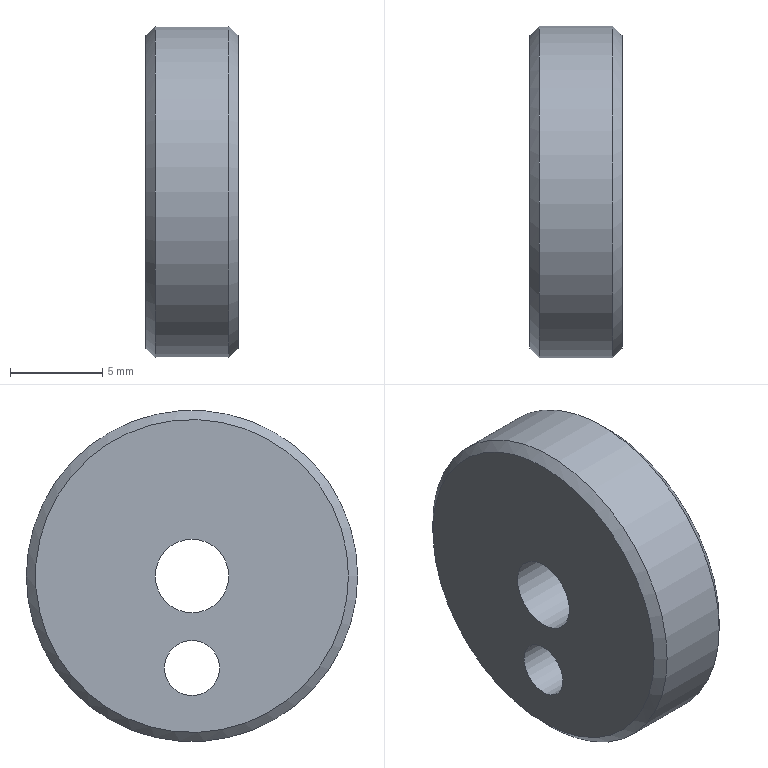Component | NX | ASSY_PRAC_PART_3 | 1 solid | 7 faces | box 5 x 18 x 18 mm | volume 1160 mm3 | cylinder 3 | plane 2 | cone 2 | commonest cylinder face diameters 3 x1 18 x1 4 x1
STEP:
#1=CARTESIAN_POINT('',(0.,0.,0.));
#2=DIRECTION('',(0.,0.,1.));
#3=DIRECTION('',(1.,0.,0.));
#4=AXIS2_PLACEMENT_3D('',#1,#2,#3);
#5=CARTESIAN_POINT('',(-8.5,-1.115,15.561));
#6=VERTEX_POINT('',#5);
#7=CARTESIAN_POINT('',(-8.5,0.3851,15.561));
#8=DIRECTION('',(-1.,0.,0.));
#9=DIRECTION('',(0.,-1.,0.));
#10=AXIS2_PLACEMENT_3D('',#7,#8,#9);
#11=CIRCLE('',#10,1.5);
#12=CARTESIAN_POINT('',(-8.5,0.3851,15.561));
#13=DIRECTION('',(-1.,0.,0.));
#14=DIRECTION('',(0.,1.,0.));
#15=AXIS2_PLACEMENT_3D('',#12,#13,#14);
#16=CYLINDRICAL_SURFACE('',#15,1.5);
#17=CARTESIAN_POINT('',(3.142,0.));
#18=DIRECTION('',(1.,0.));
#19=VECTOR('',#18,1.);
#20=LINE('',#17,#19);
#21=(GEOMETRIC_REPRESENTATION_CONTEXT(2)PARAMETRIC_REPRESENTATION_CONTEXT()REPRESENTATION_CONTEXT('',''));
#22=DEFINITIONAL_REPRESENTATION('',(#20),#21);
#23=PCURVE('',#16,#22);
#24=CARTESIAN_POINT('',(-8.5,0.3851,18.061));
#25=DIRECTION('',(1.,0.,0.));
#26=DIRECTION('',(0.,-1.,0.));
#27=AXIS2_PLACEMENT_3D('',#24,#25,#26);
#28=PLANE('',#27);
#29=CARTESIAN_POINT('',(1.5,2.5));
#30=CARTESIAN_POINT('',(1.5,-0.09808));
#31=CARTESIAN_POINT('',(-0.75,1.201));
#32=CARTESIAN_POINT('',(-3.,2.5));
#33=CARTESIAN_POINT('',(-0.75,3.799));
#34=CARTESIAN_POINT('',(1.5,5.098));
#35=CARTESIAN_POINT('',(1.5,2.5));
#36=(BOUNDED_CURVE()B_SPLINE_CURVE(2,(#29,#30,#31,#32,#33,#34,#35),.UNSPECIFIED.,.T.,.F.)B_SPLINE_CURVE_WITH_KNOTS((1,2,2,2,2,1),(-2.094,0.,2.094,4.189,6.283,8.378),.UNSPECIFIED.)CURVE()GEOMETRIC_REPRESENTATION_ITEM()RATIONAL_B_SPLINE_CURVE((1.,0.5,1.,0.5,1.,0.5,1.))REPRESENTATION_ITEM(''));
#37=(GEOMETRIC_REPRESENTATION_CONTEXT(2)PARAMETRIC_REPRESENTATION_CONTEXT()REPRESENTATION_CONTEXT('',''));
#38=DEFINITIONAL_REPRESENTATION('',(#36),#37);
#39=PCURVE('',#28,#38);
#40=SURFACE_CURVE('',#11,(#23,#39),.PCURVE_S1.);
#41=EDGE_CURVE('',#6,#6,#40,.T.);
#42=ORIENTED_EDGE('',*,*,#41,.T.);
#43=CARTESIAN_POINT('',(-13.5,-1.115,15.561));
#44=VERTEX_POINT('',#43);
#45=CARTESIAN_POINT('',(-8.5,-1.115,15.561));
#46=CARTESIAN_POINT('',(-13.5,-1.115,15.561));
#47=B_SPLINE_CURVE_WITH_KNOTS('',1,(#45,#46),.UNSPECIFIED.,.F.,.F.,(2,2),(0.,5.),.PIECEWISE_BEZIER_KNOTS.);
#48=CARTESIAN_POINT('',(9.425,0.));
#49=DIRECTION('',(0.,1.));
#50=VECTOR('',#49,1.);
#51=LINE('',#48,#50);
#52=(GEOMETRIC_REPRESENTATION_CONTEXT(2)PARAMETRIC_REPRESENTATION_CONTEXT()REPRESENTATION_CONTEXT('',''));
#53=DEFINITIONAL_REPRESENTATION('',(#51),#52);
#54=PCURVE('',#16,#53);
#55=CARTESIAN_POINT('',(3.142,0.));
#56=DIRECTION('',(0.,1.));
#57=VECTOR('',#56,1.);
#58=LINE('',#55,#57);
#59=(GEOMETRIC_REPRESENTATION_CONTEXT(2)PARAMETRIC_REPRESENTATION_CONTEXT()REPRESENTATION_CONTEXT('',''));
#60=DEFINITIONAL_REPRESENTATION('',(#58),#59);
#61=PCURVE('',#16,#60);
#62=SEAM_CURVE('',#47,(#54,#61),.PCURVE_S1.);
#63=EDGE_CURVE('',#6,#44,#62,.T.);
#64=ORIENTED_EDGE('',*,*,#63,.T.);
#65=CARTESIAN_POINT('',(-13.5,0.3851,15.561));
#66=DIRECTION('',(-1.,0.,0.));
#67=DIRECTION('',(0.,-1.,0.));
#68=AXIS2_PLACEMENT_3D('',#65,#66,#67);
#69=CIRCLE('',#68,1.5);
#70=CARTESIAN_POINT('',(3.142,5.));
#71=DIRECTION('',(1.,0.));
#72=VECTOR('',#71,1.);
#73=LINE('',#70,#72);
#74=(GEOMETRIC_REPRESENTATION_CONTEXT(2)PARAMETRIC_REPRESENTATION_CONTEXT()REPRESENTATION_CONTEXT('',''));
#75=DEFINITIONAL_REPRESENTATION('',(#73),#74);
#76=PCURVE('',#16,#75);
#77=CARTESIAN_POINT('',(-13.5,0.3851,18.061));
#78=DIRECTION('',(1.,0.,0.));
#79=DIRECTION('',(0.,-1.,0.));
#80=AXIS2_PLACEMENT_3D('',#77,#78,#79);
#81=PLANE('',#80);
#82=CARTESIAN_POINT('',(1.5,2.5));
#83=CARTESIAN_POINT('',(1.5,-0.09808));
#84=CARTESIAN_POINT('',(-0.75,1.201));
#85=CARTESIAN_POINT('',(-3.,2.5));
#86=CARTESIAN_POINT('',(-0.75,3.799));
#87=CARTESIAN_POINT('',(1.5,5.098));
#88=CARTESIAN_POINT('',(1.5,2.5));
#89=(BOUNDED_CURVE()B_SPLINE_CURVE(2,(#82,#83,#84,#85,#86,#87,#88),.UNSPECIFIED.,.T.,.F.)B_SPLINE_CURVE_WITH_KNOTS((1,2,2,2,2,1),(-2.094,0.,2.094,4.189,6.283,8.378),.UNSPECIFIED.)CURVE()GEOMETRIC_REPRESENTATION_ITEM()RATIONAL_B_SPLINE_CURVE((1.,0.5,1.,0.5,1.,0.5,1.))REPRESENTATION_ITEM(''));
#90=(GEOMETRIC_REPRESENTATION_CONTEXT(2)PARAMETRIC_REPRESENTATION_CONTEXT()REPRESENTATION_CONTEXT('',''));
#91=DEFINITIONAL_REPRESENTATION('',(#89),#90);
#92=PCURVE('',#81,#91);
#93=SURFACE_CURVE('',#69,(#76,#92),.PCURVE_S1.);
#94=EDGE_CURVE('',#44,#44,#93,.T.);
#95=ORIENTED_EDGE('',*,*,#94,.F.);
#96=ORIENTED_EDGE('',*,*,#63,.F.);
#97=EDGE_LOOP('',(#42,#64,#95,#96));
#98=FACE_BOUND('',#97,.F.);
#99=ADVANCED_FACE('',(#98),#16,.F.);
#100=CARTESIAN_POINT('',(-13.,-8.615,20.561));
#101=VERTEX_POINT('',#100);
#102=CARTESIAN_POINT('',(-13.,0.3851,20.561));
#103=DIRECTION('',(1.,0.,0.));
#104=DIRECTION('',(0.,-1.,0.));
#105=AXIS2_PLACEMENT_3D('',#102,#103,#104);
#106=CIRCLE('',#105,9.);
#107=CARTESIAN_POINT('',(-8.5,0.3851,20.561));
#108=DIRECTION('',(-1.,0.,0.));
#109=DIRECTION('',(0.,1.,0.));
#110=AXIS2_PLACEMENT_3D('',#107,#108,#109);
#111=CYLINDRICAL_SURFACE('',#110,9.);
#112=CARTESIAN_POINT('',(9.425,4.5));
#113=DIRECTION('',(-1.,0.));
#114=VECTOR('',#113,1.);
#115=LINE('',#112,#114);
#116=(GEOMETRIC_REPRESENTATION_CONTEXT(2)PARAMETRIC_REPRESENTATION_CONTEXT()REPRESENTATION_CONTEXT('',''));
#117=DEFINITIONAL_REPRESENTATION('',(#115),#116);
#118=PCURVE('',#111,#117);
#119=CARTESIAN_POINT('',(-13.5,0.3851,20.561));
#120=DIRECTION('',(1.,0.,0.));
#121=DIRECTION('',(0.,-1.,0.));
#122=AXIS2_PLACEMENT_3D('',#119,#120,#121);
#123=CONICAL_SURFACE('',#122,8.5,0.7854);
#124=CARTESIAN_POINT('',(0.,0.5));
#125=DIRECTION('',(1.,0.));
#126=VECTOR('',#125,1.);
#127=LINE('',#124,#126);
#128=(GEOMETRIC_REPRESENTATION_CONTEXT(2)PARAMETRIC_REPRESENTATION_CONTEXT()REPRESENTATION_CONTEXT('',''));
#129=DEFINITIONAL_REPRESENTATION('',(#127),#128);
#130=PCURVE('',#123,#129);
#131=SURFACE_CURVE('',#106,(#118,#130),.PCURVE_S1.);
#132=EDGE_CURVE('',#101,#101,#131,.T.);
#133=ORIENTED_EDGE('',*,*,#132,.T.);
#134=CARTESIAN_POINT('',(-9.,-8.615,20.561));
#135=VERTEX_POINT('',#134);
#136=CARTESIAN_POINT('',(-9.,-8.615,20.561));
#137=CARTESIAN_POINT('',(-13.,-8.615,20.561));
#138=B_SPLINE_CURVE_WITH_KNOTS('',1,(#136,#137),.UNSPECIFIED.,.F.,.F.,(2,2),(0.5,4.5),.PIECEWISE_BEZIER_KNOTS.);
#139=CARTESIAN_POINT('',(3.142,0.));
#140=DIRECTION('',(0.,1.));
#141=VECTOR('',#140,1.);
#142=LINE('',#139,#141);
#143=(GEOMETRIC_REPRESENTATION_CONTEXT(2)PARAMETRIC_REPRESENTATION_CONTEXT()REPRESENTATION_CONTEXT('',''));
#144=DEFINITIONAL_REPRESENTATION('',(#142),#143);
#145=PCURVE('',#111,#144);
#146=CARTESIAN_POINT('',(9.425,0.));
#147=DIRECTION('',(0.,1.));
#148=VECTOR('',#147,1.);
#149=LINE('',#146,#148);
#150=(GEOMETRIC_REPRESENTATION_CONTEXT(2)PARAMETRIC_REPRESENTATION_CONTEXT()REPRESENTATION_CONTEXT('',''));
#151=DEFINITIONAL_REPRESENTATION('',(#149),#150);
#152=PCURVE('',#111,#151);
#153=SEAM_CURVE('',#138,(#145,#152),.PCURVE_S1.);
#154=EDGE_CURVE('',#135,#101,#153,.T.);
#155=ORIENTED_EDGE('',*,*,#154,.F.);
#156=CARTESIAN_POINT('',(-9.,0.3851,20.561));
#157=DIRECTION('',(-1.,0.,0.));
#158=DIRECTION('',(0.,-1.,0.));
#159=AXIS2_PLACEMENT_3D('',#156,#157,#158);
#160=CIRCLE('',#159,9.);
#161=CARTESIAN_POINT('',(3.142,0.5));
#162=DIRECTION('',(1.,0.));
#163=VECTOR('',#162,1.);
#164=LINE('',#161,#163);
#165=(GEOMETRIC_REPRESENTATION_CONTEXT(2)PARAMETRIC_REPRESENTATION_CONTEXT()REPRESENTATION_CONTEXT('',''));
#166=DEFINITIONAL_REPRESENTATION('',(#164),#165);
#167=PCURVE('',#111,#166);
#168=CARTESIAN_POINT('',(-9.,0.3851,20.561));
#169=DIRECTION('',(-1.,0.,0.));
#170=DIRECTION('',(0.,1.,0.));
#171=AXIS2_PLACEMENT_3D('',#168,#169,#170);
#172=CONICAL_SURFACE('',#171,9.,0.7854);
#173=CARTESIAN_POINT('',(3.142,0.));
#174=DIRECTION('',(1.,0.));
#175=VECTOR('',#174,1.);
#176=LINE('',#173,#175);
#177=(GEOMETRIC_REPRESENTATION_CONTEXT(2)PARAMETRIC_REPRESENTATION_CONTEXT()REPRESENTATION_CONTEXT('',''));
#178=DEFINITIONAL_REPRESENTATION('',(#176),#177);
#179=PCURVE('',#172,#178);
#180=SURFACE_CURVE('',#160,(#167,#179),.PCURVE_S1.);
#181=EDGE_CURVE('',#135,#135,#180,.T.);
#182=ORIENTED_EDGE('',*,*,#181,.T.);
#183=ORIENTED_EDGE('',*,*,#154,.T.);
#184=EDGE_LOOP('',(#133,#155,#182,#183));
#185=FACE_BOUND('',#184,.T.);
#186=ADVANCED_FACE('',(#185),#111,.T.);
#187=CARTESIAN_POINT('',(-8.5,-1.615,20.561));
#188=VERTEX_POINT('',#187);
#189=CARTESIAN_POINT('',(-8.5,0.3851,20.561));
#190=DIRECTION('',(-1.,0.,0.));
#191=DIRECTION('',(0.,-1.,0.));
#192=AXIS2_PLACEMENT_3D('',#189,#190,#191);
#193=CIRCLE('',#192,2.);
#194=CARTESIAN_POINT('',(-8.5,0.3851,20.561));
#195=DIRECTION('',(-1.,0.,0.));
#196=DIRECTION('',(0.,1.,0.));
#197=AXIS2_PLACEMENT_3D('',#194,#195,#196);
#198=CYLINDRICAL_SURFACE('',#197,2.);
#199=CARTESIAN_POINT('',(3.142,0.));
#200=DIRECTION('',(1.,0.));
#201=VECTOR('',#200,1.);
#202=LINE('',#199,#201);
#203=(GEOMETRIC_REPRESENTATION_CONTEXT(2)PARAMETRIC_REPRESENTATION_CONTEXT()REPRESENTATION_CONTEXT('',''));
#204=DEFINITIONAL_REPRESENTATION('',(#202),#203);
#205=PCURVE('',#198,#204);
#206=CARTESIAN_POINT('',(2.,-2.5));
#207=CARTESIAN_POINT('',(2.,-5.964));
#208=CARTESIAN_POINT('',(-1.,-4.232));
#209=CARTESIAN_POINT('',(-4.,-2.5));
#210=CARTESIAN_POINT('',(-1.,-0.7679));
#211=CARTESIAN_POINT('',(2.,0.9641));
#212=CARTESIAN_POINT('',(2.,-2.5));
#213=(BOUNDED_CURVE()B_SPLINE_CURVE(2,(#206,#207,#208,#209,#210,#211,#212),.UNSPECIFIED.,.T.,.F.)B_SPLINE_CURVE_WITH_KNOTS((1,2,2,2,2,1),(-2.094,0.,2.094,4.189,6.283,8.378),.UNSPECIFIED.)CURVE()GEOMETRIC_REPRESENTATION_ITEM()RATIONAL_B_SPLINE_CURVE((1.,0.5,1.,0.5,1.,0.5,1.))REPRESENTATION_ITEM(''));
#214=(GEOMETRIC_REPRESENTATION_CONTEXT(2)PARAMETRIC_REPRESENTATION_CONTEXT()REPRESENTATION_CONTEXT('',''));
#215=DEFINITIONAL_REPRESENTATION('',(#213),#214);
#216=PCURVE('',#28,#215);
#217=SURFACE_CURVE('',#193,(#205,#216),.PCURVE_S1.);
#218=EDGE_CURVE('',#188,#188,#217,.T.);
#219=ORIENTED_EDGE('',*,*,#218,.T.);
#220=CARTESIAN_POINT('',(-13.5,-1.615,20.561));
#221=VERTEX_POINT('',#220);
#222=CARTESIAN_POINT('',(-8.5,-1.615,20.561));
#223=CARTESIAN_POINT('',(-13.5,-1.615,20.561));
#224=B_SPLINE_CURVE_WITH_KNOTS('',1,(#222,#223),.UNSPECIFIED.,.F.,.F.,(2,2),(0.,5.),.PIECEWISE_BEZIER_KNOTS.);
#225=CARTESIAN_POINT('',(9.425,0.));
#226=DIRECTION('',(0.,1.));
#227=VECTOR('',#226,1.);
#228=LINE('',#225,#227);
#229=(GEOMETRIC_REPRESENTATION_CONTEXT(2)PARAMETRIC_REPRESENTATION_CONTEXT()REPRESENTATION_CONTEXT('',''));
#230=DEFINITIONAL_REPRESENTATION('',(#228),#229);
#231=PCURVE('',#198,#230);
#232=CARTESIAN_POINT('',(3.142,0.));
#233=DIRECTION('',(0.,1.));
#234=VECTOR('',#233,1.);
#235=LINE('',#232,#234);
#236=(GEOMETRIC_REPRESENTATION_CONTEXT(2)PARAMETRIC_REPRESENTATION_CONTEXT()REPRESENTATION_CONTEXT('',''));
#237=DEFINITIONAL_REPRESENTATION('',(#235),#236);
#238=PCURVE('',#198,#237);
#239=SEAM_CURVE('',#224,(#231,#238),.PCURVE_S1.);
#240=EDGE_CURVE('',#188,#221,#239,.T.);
#241=ORIENTED_EDGE('',*,*,#240,.T.);
#242=CARTESIAN_POINT('',(-13.5,0.3851,20.561));
#243=DIRECTION('',(-1.,0.,0.));
#244=DIRECTION('',(0.,-1.,0.));
#245=AXIS2_PLACEMENT_3D('',#242,#243,#244);
#246=CIRCLE('',#245,2.);
#247=CARTESIAN_POINT('',(3.142,5.));
#248=DIRECTION('',(1.,0.));
#249=VECTOR('',#248,1.);
#250=LINE('',#247,#249);
#251=(GEOMETRIC_REPRESENTATION_CONTEXT(2)PARAMETRIC_REPRESENTATION_CONTEXT()REPRESENTATION_CONTEXT('',''));
#252=DEFINITIONAL_REPRESENTATION('',(#250),#251);
#253=PCURVE('',#198,#252);
#254=CARTESIAN_POINT('',(2.,-2.5));
#255=CARTESIAN_POINT('',(2.,-5.964));
#256=CARTESIAN_POINT('',(-1.,-4.232));
#257=CARTESIAN_POINT('',(-4.,-2.5));
#258=CARTESIAN_POINT('',(-1.,-0.7679));
#259=CARTESIAN_POINT('',(2.,0.9641));
#260=CARTESIAN_POINT('',(2.,-2.5));
#261=(BOUNDED_CURVE()B_SPLINE_CURVE(2,(#254,#255,#256,#257,#258,#259,#260),.UNSPECIFIED.,.T.,.F.)B_SPLINE_CURVE_WITH_KNOTS((1,2,2,2,2,1),(-2.094,0.,2.094,4.189,6.283,8.378),.UNSPECIFIED.)CURVE()GEOMETRIC_REPRESENTATION_ITEM()RATIONAL_B_SPLINE_CURVE((1.,0.5,1.,0.5,1.,0.5,1.))REPRESENTATION_ITEM(''));
#262=(GEOMETRIC_REPRESENTATION_CONTEXT(2)PARAMETRIC_REPRESENTATION_CONTEXT()REPRESENTATION_CONTEXT('',''));
#263=DEFINITIONAL_REPRESENTATION('',(#261),#262);
#264=PCURVE('',#81,#263);
#265=SURFACE_CURVE('',#246,(#253,#264),.PCURVE_S1.);
#266=EDGE_CURVE('',#221,#221,#265,.T.);
#267=ORIENTED_EDGE('',*,*,#266,.F.);
#268=ORIENTED_EDGE('',*,*,#240,.F.);
#269=EDGE_LOOP('',(#219,#241,#267,#268));
#270=FACE_BOUND('',#269,.F.);
#271=ADVANCED_FACE('',(#270),#198,.F.);
#272=CARTESIAN_POINT('',(-8.5,-8.115,20.561));
#273=VERTEX_POINT('',#272);
#274=CARTESIAN_POINT('',(-8.5,0.3851,20.561));
#275=DIRECTION('',(1.,0.,0.));
#276=DIRECTION('',(0.,-1.,0.));
#277=AXIS2_PLACEMENT_3D('',#274,#275,#276);
#278=CIRCLE('',#277,8.5);
#279=CARTESIAN_POINT('',(0.,-2.5));
#280=DIRECTION('',(1.,0.));
#281=AXIS2_PLACEMENT_2D('',#279,#280);
#282=CIRCLE('',#281,8.5);
#283=(GEOMETRIC_REPRESENTATION_CONTEXT(2)PARAMETRIC_REPRESENTATION_CONTEXT()REPRESENTATION_CONTEXT('',''));
#284=DEFINITIONAL_REPRESENTATION('',(#282),#283);
#285=PCURVE('',#28,#284);
#286=CARTESIAN_POINT('',(9.425,-0.5));
#287=DIRECTION('',(-1.,0.));
#288=VECTOR('',#287,1.);
#289=LINE('',#286,#288);
#290=(GEOMETRIC_REPRESENTATION_CONTEXT(2)PARAMETRIC_REPRESENTATION_CONTEXT()REPRESENTATION_CONTEXT('',''));
#291=DEFINITIONAL_REPRESENTATION('',(#289),#290);
#292=PCURVE('',#172,#291);
#293=SURFACE_CURVE('',#278,(#285,#292),.PCURVE_S1.);
#294=EDGE_CURVE('',#273,#273,#293,.T.);
#295=ORIENTED_EDGE('',*,*,#294,.T.);
#296=EDGE_LOOP('',(#295));
#297=FACE_BOUND('',#296,.T.);
#298=ORIENTED_EDGE('',*,*,#41,.T.);
#299=EDGE_LOOP('',(#298));
#300=FACE_BOUND('',#299,.T.);
#301=ORIENTED_EDGE('',*,*,#218,.T.);
#302=EDGE_LOOP('',(#301));
#303=FACE_BOUND('',#302,.T.);
#304=ADVANCED_FACE('',(#297,#300,#303),#28,.T.);
#305=CARTESIAN_POINT('',(-13.5,-8.115,20.561));
#306=VERTEX_POINT('',#305);
#307=CARTESIAN_POINT('',(-13.5,0.3851,20.561));
#308=DIRECTION('',(-1.,0.,0.));
#309=DIRECTION('',(0.,-1.,0.));
#310=AXIS2_PLACEMENT_3D('',#307,#308,#309);
#311=CIRCLE('',#310,8.5);
#312=CARTESIAN_POINT('',(8.5,-2.5));
#313=CARTESIAN_POINT('',(8.5,-17.222));
#314=CARTESIAN_POINT('',(-4.25,-9.861));
#315=CARTESIAN_POINT('',(-17.,-2.5));
#316=CARTESIAN_POINT('',(-4.25,4.861));
#317=CARTESIAN_POINT('',(8.5,12.222));
#318=CARTESIAN_POINT('',(8.5,-2.5));
#319=(BOUNDED_CURVE()B_SPLINE_CURVE(2,(#312,#313,#314,#315,#316,#317,#318),.UNSPECIFIED.,.T.,.F.)B_SPLINE_CURVE_WITH_KNOTS((1,2,2,2,2,1),(-2.094,0.,2.094,4.189,6.283,8.378),.UNSPECIFIED.)CURVE()GEOMETRIC_REPRESENTATION_ITEM()RATIONAL_B_SPLINE_CURVE((1.,0.5,1.,0.5,1.,0.5,1.))REPRESENTATION_ITEM(''));
#320=(GEOMETRIC_REPRESENTATION_CONTEXT(2)PARAMETRIC_REPRESENTATION_CONTEXT()REPRESENTATION_CONTEXT('',''));
#321=DEFINITIONAL_REPRESENTATION('',(#319),#320);
#322=PCURVE('',#81,#321);
#323=CARTESIAN_POINT('',(6.283,0.));
#324=DIRECTION('',(-1.,0.));
#325=VECTOR('',#324,1.);
#326=LINE('',#323,#325);
#327=(GEOMETRIC_REPRESENTATION_CONTEXT(2)PARAMETRIC_REPRESENTATION_CONTEXT()REPRESENTATION_CONTEXT('',''));
#328=DEFINITIONAL_REPRESENTATION('',(#326),#327);
#329=PCURVE('',#123,#328);
#330=SURFACE_CURVE('',#311,(#322,#329),.PCURVE_S1.);
#331=EDGE_CURVE('',#306,#306,#330,.T.);
#332=ORIENTED_EDGE('',*,*,#331,.T.);
#333=EDGE_LOOP('',(#332));
#334=FACE_BOUND('',#333,.T.);
#335=ORIENTED_EDGE('',*,*,#94,.F.);
#336=EDGE_LOOP('',(#335));
#337=FACE_BOUND('',#336,.T.);
#338=ORIENTED_EDGE('',*,*,#266,.F.);
#339=EDGE_LOOP('',(#338));
#340=FACE_BOUND('',#339,.T.);
#341=ADVANCED_FACE('',(#334,#337,#340),#81,.F.);
#342=ORIENTED_EDGE('',*,*,#132,.F.);
#343=CARTESIAN_POINT('',(-13.5,-8.115,20.561));
#344=CARTESIAN_POINT('',(-13.,-8.615,20.561));
#345=B_SPLINE_CURVE_WITH_KNOTS('',1,(#343,#344),.UNSPECIFIED.,.F.,.F.,(2,2),(0.,0.7071),.PIECEWISE_BEZIER_KNOTS.);
#346=CARTESIAN_POINT('',(0.,0.));
#347=DIRECTION('',(0.,1.));
#348=VECTOR('',#347,1.);
#349=LINE('',#346,#348);
#350=(GEOMETRIC_REPRESENTATION_CONTEXT(2)PARAMETRIC_REPRESENTATION_CONTEXT()REPRESENTATION_CONTEXT('',''));
#351=DEFINITIONAL_REPRESENTATION('',(#349),#350);
#352=PCURVE('',#123,#351);
#353=CARTESIAN_POINT('',(6.283,0.));
#354=DIRECTION('',(0.,1.));
#355=VECTOR('',#354,1.);
#356=LINE('',#353,#355);
#357=(GEOMETRIC_REPRESENTATION_CONTEXT(2)PARAMETRIC_REPRESENTATION_CONTEXT()REPRESENTATION_CONTEXT('',''));
#358=DEFINITIONAL_REPRESENTATION('',(#356),#357);
#359=PCURVE('',#123,#358);
#360=SEAM_CURVE('',#345,(#352,#359),.PCURVE_S1.);
#361=EDGE_CURVE('',#306,#101,#360,.T.);
#362=ORIENTED_EDGE('',*,*,#361,.F.);
#363=ORIENTED_EDGE('',*,*,#331,.F.);
#364=ORIENTED_EDGE('',*,*,#361,.T.);
#365=EDGE_LOOP('',(#342,#362,#363,#364));
#366=FACE_BOUND('',#365,.T.);
#367=ADVANCED_FACE('',(#366),#123,.T.);
#368=ORIENTED_EDGE('',*,*,#294,.F.);
#369=CARTESIAN_POINT('',(-8.5,-8.115,20.561));
#370=CARTESIAN_POINT('',(-9.,-8.615,20.561));
#371=B_SPLINE_CURVE_WITH_KNOTS('',1,(#369,#370),.UNSPECIFIED.,.F.,.F.,(2,2),(-0.7071,0.),.PIECEWISE_BEZIER_KNOTS.);
#372=CARTESIAN_POINT('',(9.425,0.));
#373=DIRECTION('',(0.,1.));
#374=VECTOR('',#373,1.);
#375=LINE('',#372,#374);
#376=(GEOMETRIC_REPRESENTATION_CONTEXT(2)PARAMETRIC_REPRESENTATION_CONTEXT()REPRESENTATION_CONTEXT('',''));
#377=DEFINITIONAL_REPRESENTATION('',(#375),#376);
#378=PCURVE('',#172,#377);
#379=CARTESIAN_POINT('',(3.142,0.));
#380=DIRECTION('',(0.,1.));
#381=VECTOR('',#380,1.);
#382=LINE('',#379,#381);
#383=(GEOMETRIC_REPRESENTATION_CONTEXT(2)PARAMETRIC_REPRESENTATION_CONTEXT()REPRESENTATION_CONTEXT('',''));
#384=DEFINITIONAL_REPRESENTATION('',(#382),#383);
#385=PCURVE('',#172,#384);
#386=SEAM_CURVE('',#371,(#378,#385),.PCURVE_S1.);
#387=EDGE_CURVE('',#273,#135,#386,.T.);
#388=ORIENTED_EDGE('',*,*,#387,.T.);
#389=ORIENTED_EDGE('',*,*,#181,.F.);
#390=ORIENTED_EDGE('',*,*,#387,.F.);
#391=EDGE_LOOP('',(#368,#388,#389,#390));
#392=FACE_BOUND('',#391,.T.);
#393=ADVANCED_FACE('',(#392),#172,.T.);
#394=CLOSED_SHELL('',(#99,#186,#271,#304,#341,#367,#393));
#395=MANIFOLD_SOLID_BREP('',#394);
#396=(LENGTH_UNIT()NAMED_UNIT(*)SI_UNIT(.MILLI.,.METRE.));
#397=UNCERTAINTY_MEASURE_WITH_UNIT(LENGTH_MEASURE(0.00001),#396,'','');
#398=(NAMED_UNIT(*)PLANE_ANGLE_UNIT()SI_UNIT($,.RADIAN.));
#399=(NAMED_UNIT(*)SI_UNIT($,.STERADIAN.)SOLID_ANGLE_UNIT());
#400=(GEOMETRIC_REPRESENTATION_CONTEXT(3)GLOBAL_UNCERTAINTY_ASSIGNED_CONTEXT((#397))GLOBAL_UNIT_ASSIGNED_CONTEXT((#396,#398,#399))REPRESENTATION_CONTEXT('',''));
#401=ADVANCED_BREP_SHAPE_REPRESENTATION('',(#4,#395),#400);